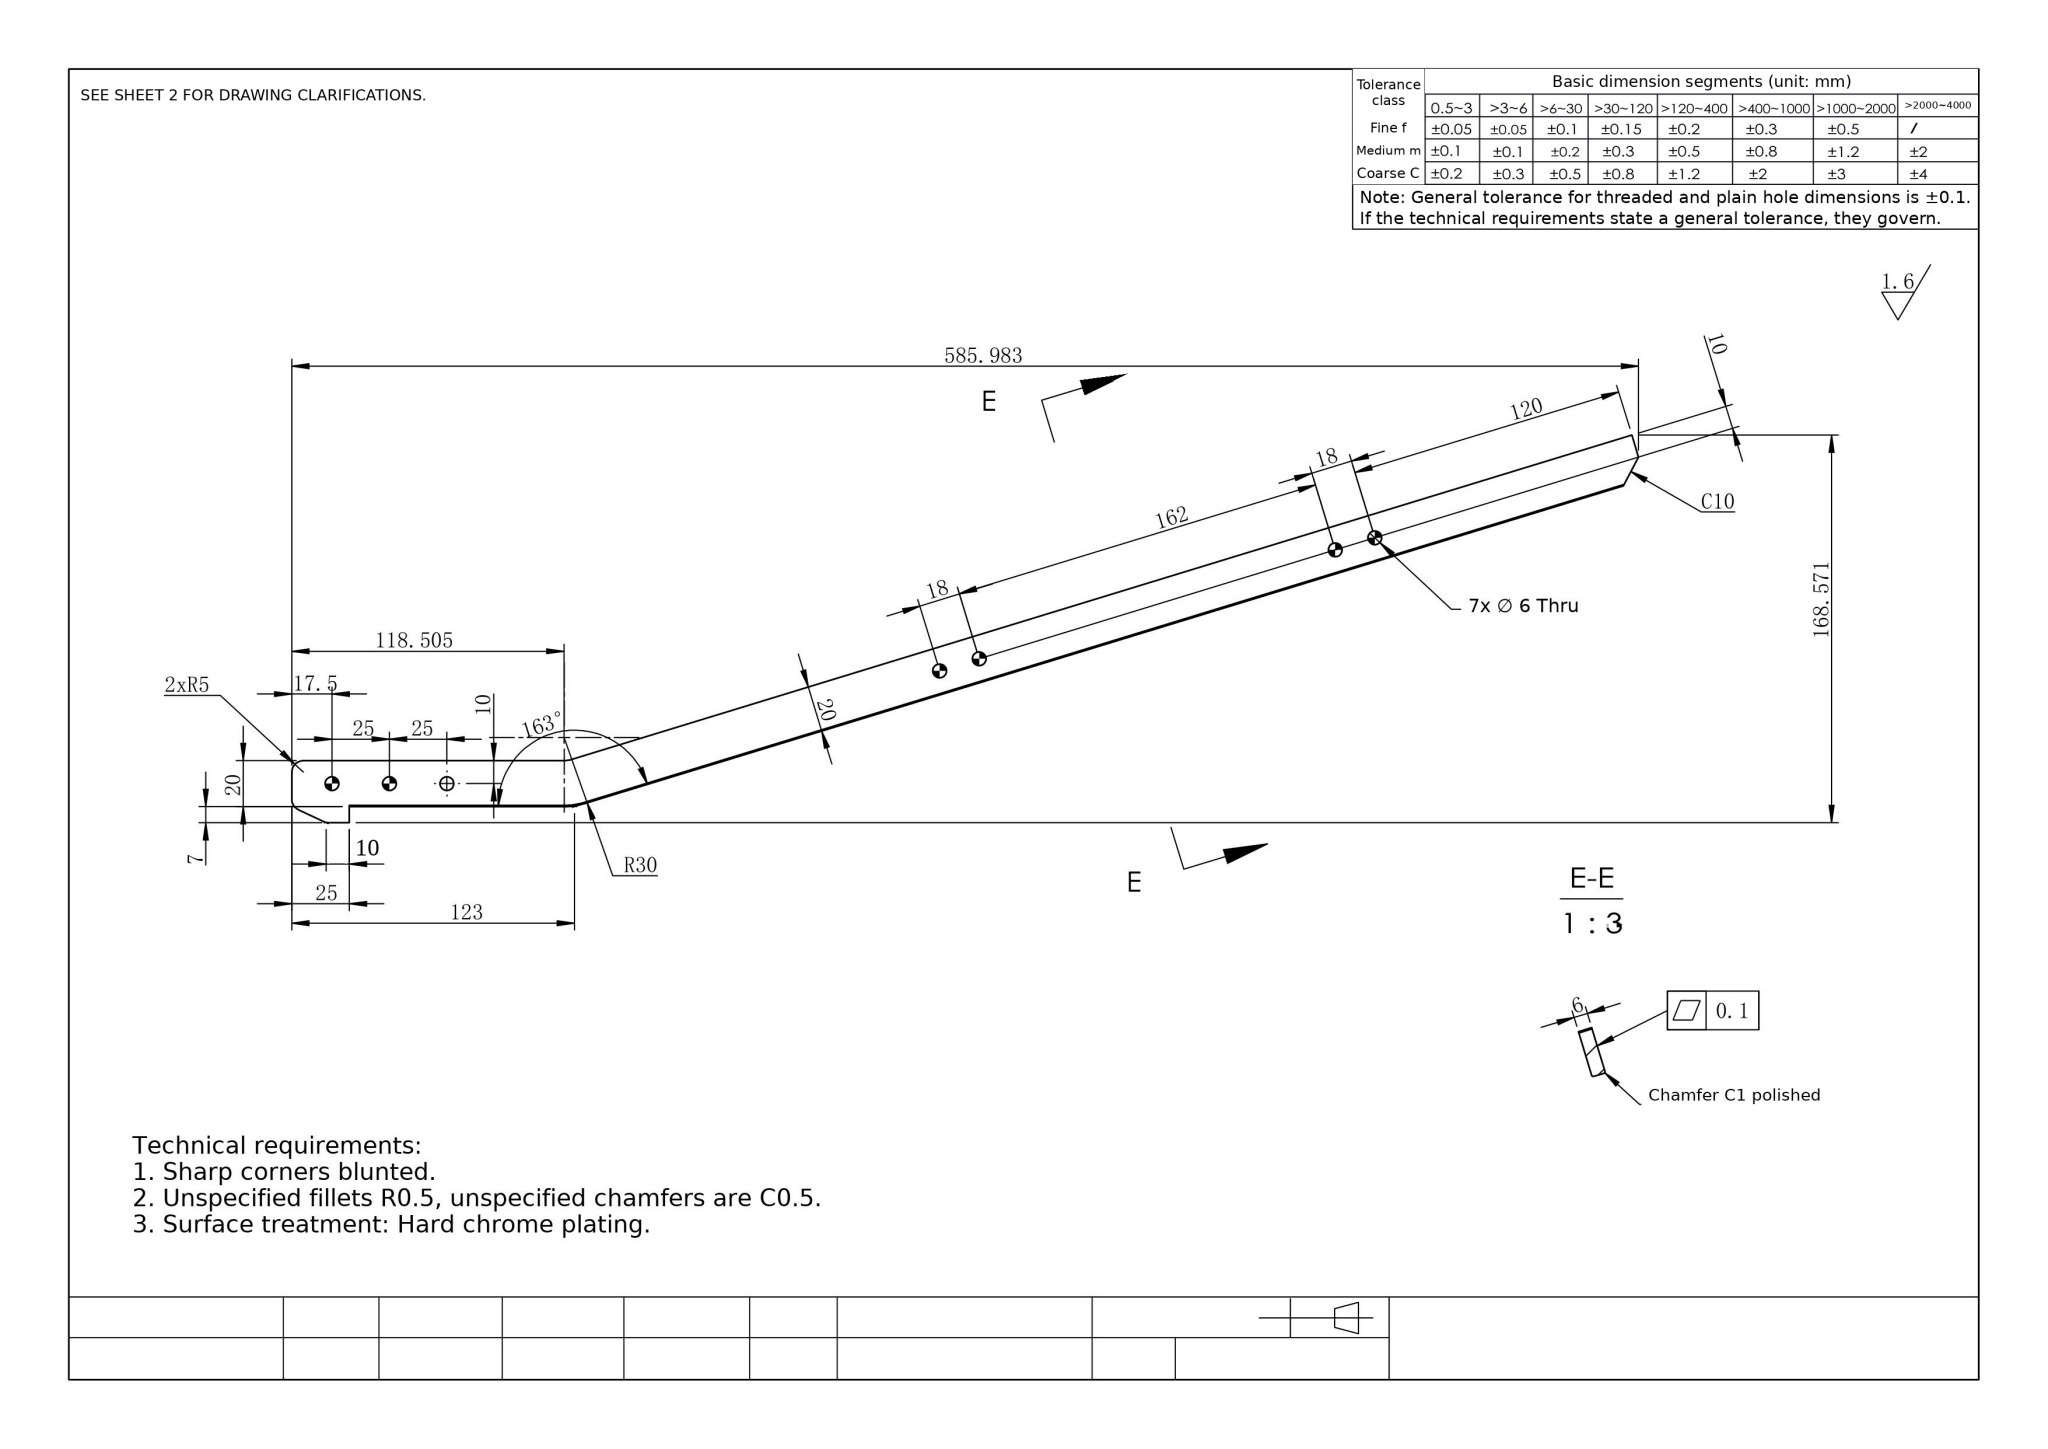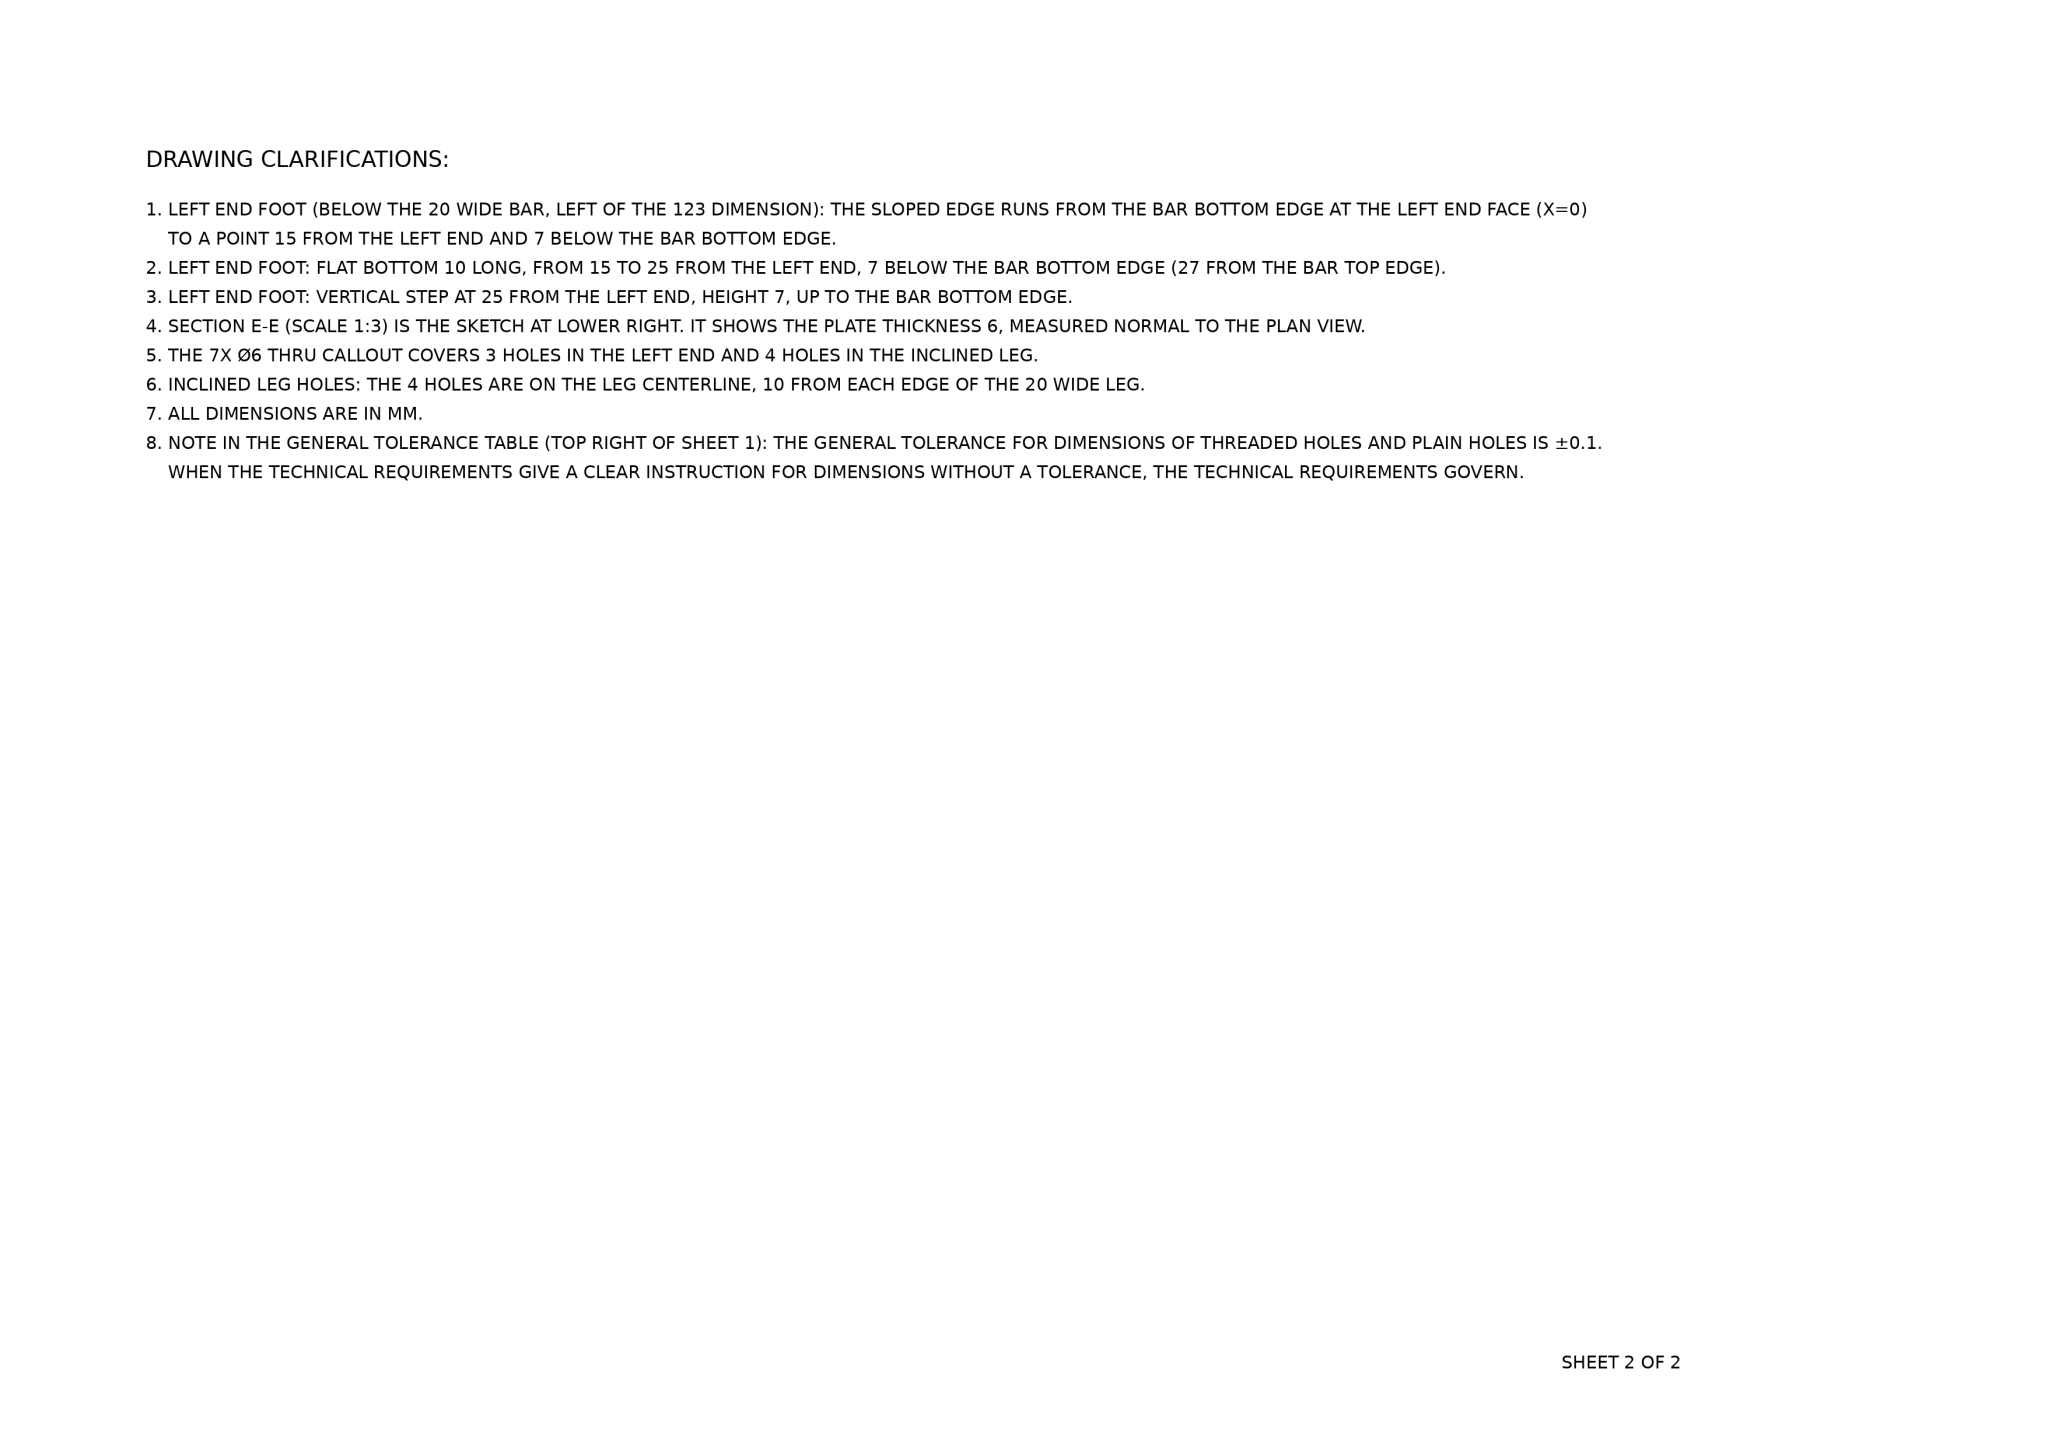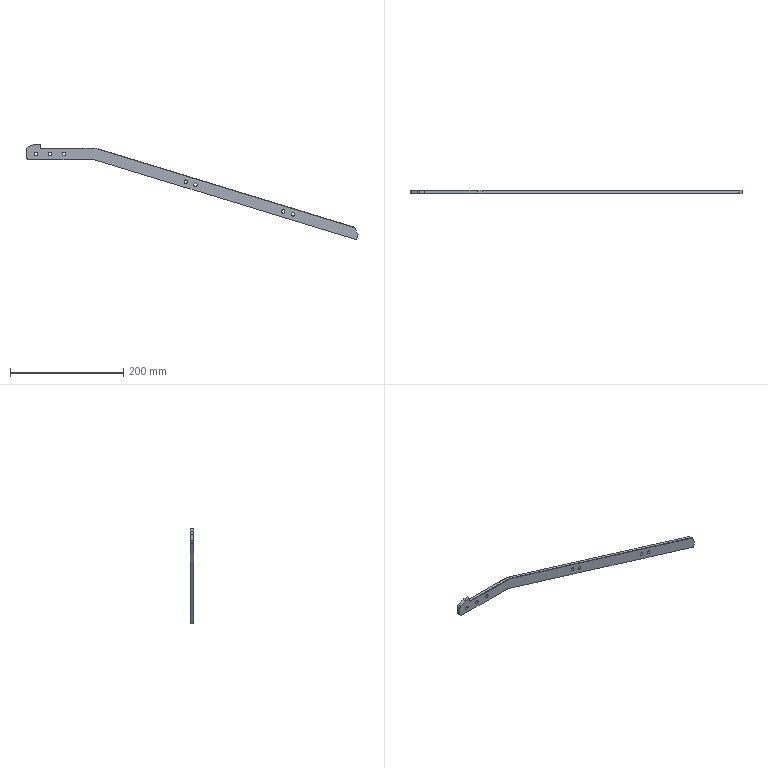Part | NX | mm | 1 solid | 37 faces | box 585.98 x 6 x 168.57 mm | volume 71920 mm3 | cylinder 19 | plane 16 | cone 2 | commonest cylinder face diameters 6 x14 10 x3 20 x1 60 x1